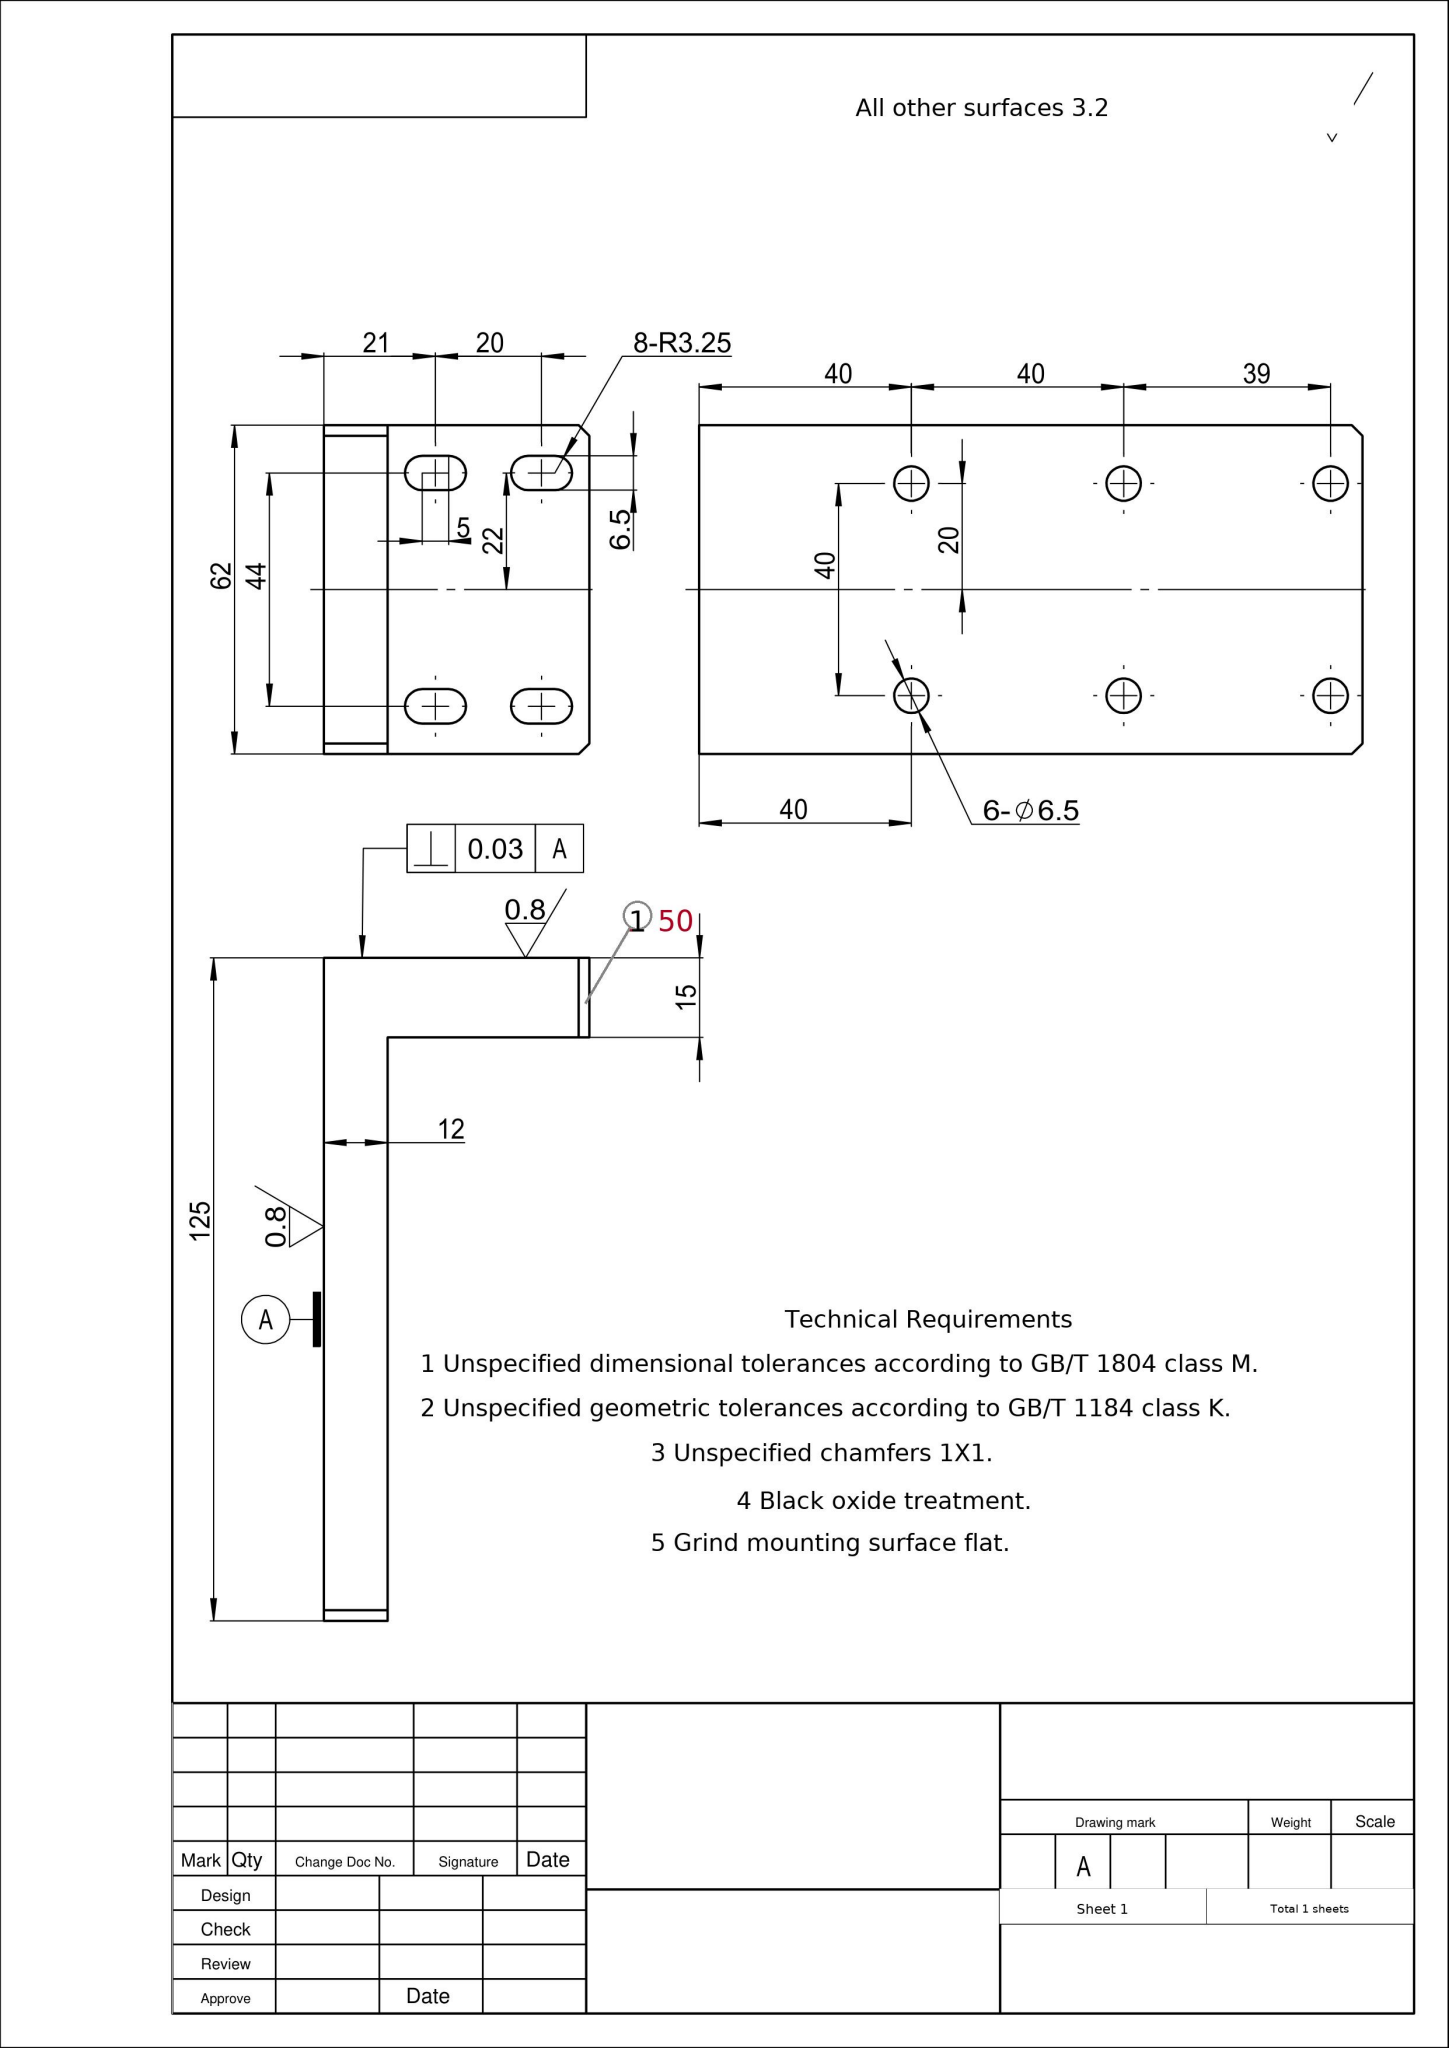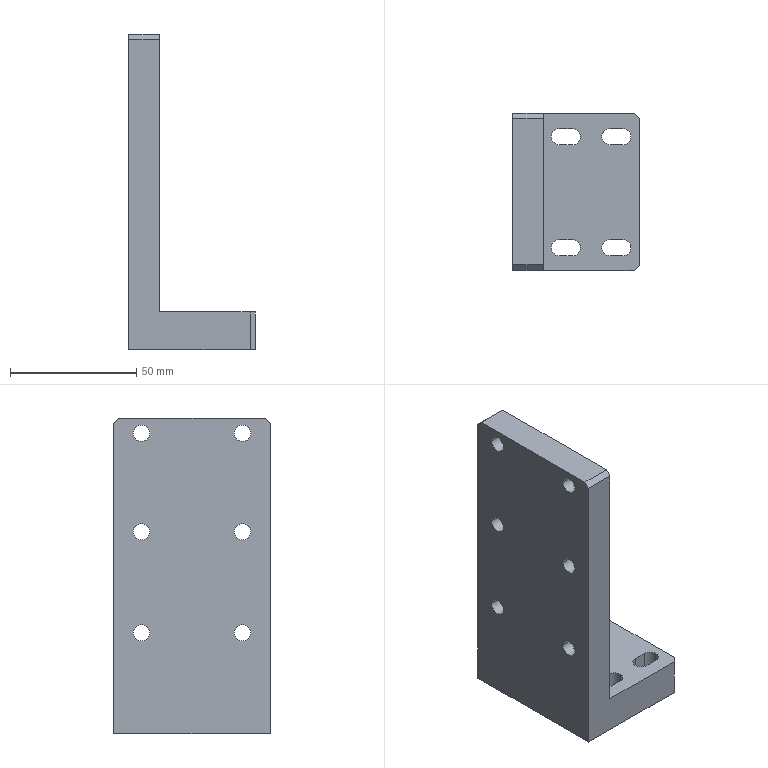Part | SolidWorks | mm | 1 solid | 44 faces | box 50 x 62 x 125 mm | volume 121902 mm3 | cylinder 24 | plane 20 | commonest cylinder face diameters 6.5 x24
build123d program:
from build123d import *

# Parameters (mm, degrees)
SKETCH1_W           = 50
SKETCH1_H           = 62
BOSS_EXTRUDE1_DEPTH = 15
SKETCH2_W           = 12
SKETCH2_H           = 62
BOSS_EXTRUDE2_DEPTH = 110
CUT_EXTRUDE1_DEPTH  = 136.809
SKETCH4_R           = 3.25
CUT_EXTRUDE2_DEPTH  = 145.613
CHAMFER1_SIZE       = 2
SKETCH5_R           = 3.25
CUT_EXTRUDE3_DEPTH  = 145.613


with BuildPart() as part:
    # Sketch1 → Boss-Extrude1 (new body)
    with BuildSketch(Plane.XY):
        with Locations((25, -31)):
            Rectangle(SKETCH1_W, SKETCH1_H)
    extrude(amount=BOSS_EXTRUDE1_DEPTH)

    # Sketch2 → Boss-Extrude2 (add)
    with BuildSketch(Plane.XY.offset(15)):
        with Locations((6, -31)):
            Rectangle(SKETCH2_W, SKETCH2_H)
    extrude(amount=BOSS_EXTRUDE2_DEPTH)

    # Sketch3 → Cut-Extrude1 (cut, through all)
    with BuildSketch(Plane.XY.offset(15)):
        with BuildLine():
            Line((18.5, -5.75), (23.5, -5.75))
            ThreePointArc((23.5, -5.75), (26.75, -9), (23.5, -12.25))
            Line((23.5, -12.25), (18.5, -12.25))
            ThreePointArc((18.5, -12.25), (15.25, -9), (18.5, -5.75))
        make_face()
        with BuildLine():
            Line((43.5, -5.75), (38.5, -5.75))
            ThreePointArc((38.5, -5.75), (35.25, -9), (38.5, -12.25))
            Line((38.5, -12.25), (43.5, -12.25))
            ThreePointArc((43.5, -12.25), (46.75, -9), (43.5, -5.75))
        make_face()
        with BuildLine():
            Line((43.5, -56.25), (38.5, -56.25))
            ThreePointArc((38.5, -56.25), (35.25, -53), (38.5, -49.75))
            Line((38.5, -49.75), (43.5, -49.75))
            ThreePointArc((43.5, -49.75), (46.75, -53), (43.5, -56.25))
        make_face()
        with BuildLine():
            Line((18.5, -56.25), (23.5, -56.25))
            ThreePointArc((23.5, -56.25), (26.75, -53), (23.5, -49.75))
            Line((23.5, -49.75), (18.5, -49.75))
            ThreePointArc((18.5, -49.75), (15.25, -53), (18.5, -56.25))
        make_face()
    extrude(amount=-CUT_EXTRUDE1_DEPTH, mode=Mode.SUBTRACT)

    # Sketch4 → Cut-Extrude2 (cut, through all)
    with BuildSketch(Plane(origin=(12, 0, 0), x_dir=(0, 0, -1), z_dir=(1, 0, 0))):
        with Locations(Location((-80, -11, 0), (0, 0, 90))):
            Circle(SKETCH4_R)
        with Locations(Location((-40, -11, 0), (0, 0, 90))):
            Circle(SKETCH4_R)
        with Locations(Location((-40, -51, 0), (0, 0, 270))):
            Circle(SKETCH4_R)
        with Locations(Location((-80, -51, 0), (0, 0, 270))):
            Circle(SKETCH4_R)
    extrude(amount=-CUT_EXTRUDE2_DEPTH, mode=Mode.SUBTRACT)

    # Chamfer1
    chamfer1_edges = [part.edges().sort_by_distance(p)[0] for p in [
        (50, 0, 7.5),
        (50, -62, 7.5),
        (6, -62, 125),
        (6, 0, 125),
    ]]
    chamfer(chamfer1_edges, length=CHAMFER1_SIZE)

    # Sketch5 → Cut-Extrude3 (cut, through all)
    with BuildSketch(Plane(origin=(12, 0, 0), x_dir=(0, 0, -1), z_dir=(1, 0, 0))):
        with Locations(Location((-119, -51, 0), (0, 0, 90))):
            Circle(SKETCH5_R)
        with Locations(Location((-119, -11, 0), (0, 0, 90))):
            Circle(SKETCH5_R)
    extrude(amount=-CUT_EXTRUDE3_DEPTH, mode=Mode.SUBTRACT)


solid = part.part